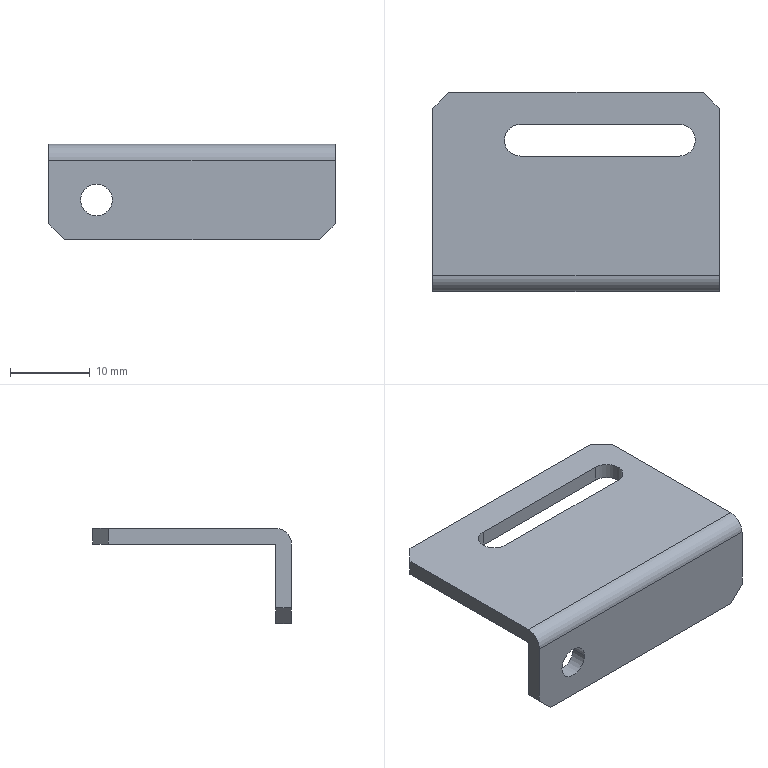Component | SolidWorks | WirePressingUnitFiberOpticBracket-1 | 1 solid | 20 faces | box 36 x 25 x 12 mm | volume 2263 mm3 | plane 14 | cylinder 6 | commonest cylinder face diameters 4 x6
build123d program:
from build123d import *

# Parameters (mm, degrees)
BOSS_EXTRUDE1_DEPTH = 18
M4_TAPPED_HOLE1_D   = 4
CHAMFER1_SIZE       = 2
CUT_EXTRUDE1_DEPTH  = 10


with BuildPart() as part:
    # Sketch1 → Boss-Extrude1 (new, symmetric)
    with BuildSketch(Plane.XY):
        with BuildLine():
            Line((0, 0), (10, 0))
            ThreePointArc((10, 0), (11.414, 0.5858), (12, 2))
            Line((12, 2), (12, 25))
            Line((12, 25), (10, 25))
            Line((10, 25), (10, 2))
            Line((10, 2), (0, 2))
            Line((0, 2), (0, 0))
        make_face()
    extrude(amount=BOSS_EXTRUDE1_DEPTH, both=True)

    # M4 Tapped Hole1 (through all)
    with Locations(Plane(origin=(0, 0, 0), x_dir=(-1, 0, 0), z_dir=(0, -1, 0))):
        with Locations((-5, -12)):
            Hole(M4_TAPPED_HOLE1_D / 2)

    # Chamfer1
    chamfer1_edges = [part.edges().sort_by_distance(p)[0] for p in [
        (11, 25, 18),
        (0, 1, 18),
        (11, 25, -18),
        (0, 1, -18),
    ]]
    chamfer(chamfer1_edges, length=CHAMFER1_SIZE)

    # Sketch4 → Cut-Extrude1 (cut)
    with BuildSketch(Plane.ZY.offset(-10)):
        with BuildLine():
            Line((-13, 21), (7, 21))
            ThreePointArc((7, 21), (9, 19), (7, 17))
            Line((7, 17), (-13, 17))
            ThreePointArc((-13, 17), (-15, 19), (-13, 21))
        make_face()
    extrude(amount=-CUT_EXTRUDE1_DEPTH, mode=Mode.SUBTRACT)


solid = part.part

# Placed as in the assembly
solid = solid.moved(Location((32.665, -6.632, -220.315), (0, -90, 0)))
STEP:
#1=COLOUR_RGB('',0.7922,0.8196,0.9333);
#2=FILL_AREA_STYLE_COLOUR('',#1);
#3=FILL_AREA_STYLE('',(#2));
#4=SURFACE_STYLE_FILL_AREA(#3);
#5=SURFACE_SIDE_STYLE('',(#4));
#6=SURFACE_STYLE_USAGE(.BOTH.,#5);
#7=PRESENTATION_STYLE_ASSIGNMENT((#6));
#8=CARTESIAN_POINT('',(0.9317,0.4869,-8.201));
#9=VERTEX_POINT('',#8);
#10=CARTESIAN_POINT('',(1.01,0.5657,-8.201));
#11=VERTEX_POINT('',#10);
#12=CARTESIAN_POINT('',(1.01,0.4869,-8.201));
#13=DIRECTION('',(-0.,0.,-1.));
#14=DIRECTION('',(0.,-1.,0.));
#15=AXIS2_PLACEMENT_3D('',#12,#13,#14);
#16=CIRCLE('',#15,0.07874);
#17=EDGE_CURVE('',#9,#11,#16,.T.);
#18=ORIENTED_EDGE('',*,*,#17,.F.);
#19=CARTESIAN_POINT('',(0.9317,0.4869,-8.28));
#20=VERTEX_POINT('',#19);
#21=CARTESIAN_POINT('',(0.9317,0.4869,-7.886));
#22=DIRECTION('',(-0.,-0.,-1.));
#23=VECTOR('',#22,39.37);
#24=LINE('',#21,#23);
#25=EDGE_CURVE('',#9,#20,#24,.T.);
#26=ORIENTED_EDGE('',*,*,#25,.T.);
#27=CARTESIAN_POINT('',(1.01,0.5657,-8.28));
#28=VERTEX_POINT('',#27);
#29=CARTESIAN_POINT('',(1.01,0.4869,-8.28));
#30=DIRECTION('',(-0.,-0.,-1.));
#31=DIRECTION('',(-1.,0.,0.));
#32=AXIS2_PLACEMENT_3D('',#29,#30,#31);
#33=CIRCLE('',#32,0.07874);
#34=EDGE_CURVE('',#20,#28,#33,.T.);
#35=ORIENTED_EDGE('',*,*,#34,.T.);
#36=CARTESIAN_POINT('',(1.01,0.5657,-7.886));
#37=DIRECTION('',(-0.,-0.,-1.));
#38=VECTOR('',#37,39.37);
#39=LINE('',#36,#38);
#40=EDGE_CURVE('',#11,#28,#39,.T.);
#41=ORIENTED_EDGE('',*,*,#40,.F.);
#42=EDGE_LOOP('',(#18,#26,#35,#41));
#43=FACE_OUTER_BOUND('',#42,.T.);
#44=CARTESIAN_POINT('',(1.01,0.4869,-7.886));
#45=DIRECTION('',(-0.,-0.,-1.));
#46=DIRECTION('',(-1.,0.,0.));
#47=AXIS2_PLACEMENT_3D('',#44,#45,#46);
#48=CYLINDRICAL_SURFACE('',#47,0.07874);
#49=ADVANCED_FACE('',(#43),#48,.F.);
#50=CARTESIAN_POINT('',(0.7348,-0.1824,-8.477));
#51=VERTEX_POINT('',#50);
#52=CARTESIAN_POINT('',(0.8923,-0.1824,-8.477));
#53=VERTEX_POINT('',#52);
#54=CARTESIAN_POINT('',(0.8136,-0.1824,-8.477));
#55=DIRECTION('',(-0.,-1.,-0.));
#56=DIRECTION('',(1.,0.,0.));
#57=AXIS2_PLACEMENT_3D('',#54,#55,#56);
#58=CIRCLE('',#57,0.07874);
#59=EDGE_CURVE('',#51,#53,#58,.T.);
#60=ORIENTED_EDGE('',*,*,#59,.F.);
#61=CARTESIAN_POINT('',(0.7348,-0.2611,-8.477));
#62=VERTEX_POINT('',#61);
#63=CARTESIAN_POINT('',(0.7348,-0.2611,-8.477));
#64=DIRECTION('',(-0.,-1.,-0.));
#65=VECTOR('',#64,39.37);
#66=LINE('',#63,#65);
#67=EDGE_CURVE('',#51,#62,#66,.T.);
#68=ORIENTED_EDGE('',*,*,#67,.T.);
#69=CARTESIAN_POINT('',(0.8923,-0.2611,-8.477));
#70=VERTEX_POINT('',#69);
#71=CARTESIAN_POINT('',(0.8136,-0.2611,-8.477));
#72=DIRECTION('',(-0.,-1.,-0.));
#73=DIRECTION('',(1.,0.,0.));
#74=AXIS2_PLACEMENT_3D('',#71,#72,#73);
#75=CIRCLE('',#74,0.07874);
#76=EDGE_CURVE('',#62,#70,#75,.T.);
#77=ORIENTED_EDGE('',*,*,#76,.T.);
#78=CARTESIAN_POINT('',(0.8923,-0.2611,-8.477));
#79=DIRECTION('',(-0.,-1.,-0.));
#80=VECTOR('',#79,39.37);
#81=LINE('',#78,#80);
#82=EDGE_CURVE('',#53,#70,#81,.T.);
#83=ORIENTED_EDGE('',*,*,#82,.F.);
#84=EDGE_LOOP('',(#60,#68,#77,#83));
#85=FACE_OUTER_BOUND('',#84,.T.);
#86=CARTESIAN_POINT('',(0.8136,-0.2611,-8.477));
#87=DIRECTION('',(-0.,-1.,-0.));
#88=DIRECTION('',(1.,0.,0.));
#89=AXIS2_PLACEMENT_3D('',#86,#87,#88);
#90=CYLINDRICAL_SURFACE('',#89,0.07874);
#91=ADVANCED_FACE('',(#85),#90,.F.);
#92=CARTESIAN_POINT('',(0.6561,-0.1824,-8.674));
#93=VERTEX_POINT('',#92);
#94=CARTESIAN_POINT('',(1.916,-0.1824,-8.674));
#95=VERTEX_POINT('',#94);
#96=CARTESIAN_POINT('',(0.5774,-0.1824,-8.674));
#97=DIRECTION('',(1.,0.,-0.));
#98=VECTOR('',#97,39.37);
#99=LINE('',#96,#98);
#100=EDGE_CURVE('',#93,#95,#99,.T.);
#101=ORIENTED_EDGE('',*,*,#100,.T.);
#102=CARTESIAN_POINT('',(1.916,-0.2611,-8.674));
#103=VERTEX_POINT('',#102);
#104=CARTESIAN_POINT('',(1.916,-0.1824,-8.674));
#105=DIRECTION('',(-0.,-1.,-0.));
#106=VECTOR('',#105,39.37);
#107=LINE('',#104,#106);
#108=EDGE_CURVE('',#95,#103,#107,.T.);
#109=ORIENTED_EDGE('',*,*,#108,.T.);
#110=CARTESIAN_POINT('',(0.6561,-0.2611,-8.674));
#111=VERTEX_POINT('',#110);
#112=CARTESIAN_POINT('',(0.5774,-0.2611,-8.674));
#113=DIRECTION('',(1.,0.,-0.));
#114=VECTOR('',#113,39.37);
#115=LINE('',#112,#114);
#116=EDGE_CURVE('',#111,#103,#115,.T.);
#117=ORIENTED_EDGE('',*,*,#116,.F.);
#118=CARTESIAN_POINT('',(0.6561,-0.1824,-8.674));
#119=DIRECTION('',(0.,1.,0.));
#120=VECTOR('',#119,39.37);
#121=LINE('',#118,#120);
#122=EDGE_CURVE('',#111,#93,#121,.T.);
#123=ORIENTED_EDGE('',*,*,#122,.T.);
#124=EDGE_LOOP('',(#101,#109,#117,#123));
#125=FACE_OUTER_BOUND('',#124,.T.);
#126=CARTESIAN_POINT('',(0.5774,-0.1824,-8.674));
#127=DIRECTION('',(0.,0.,1.));
#128=DIRECTION('',(1.,0.,-0.));
#129=AXIS2_PLACEMENT_3D('',#126,#127,#128);
#130=PLANE('',#129);
#131=ADVANCED_FACE('',(#125),#130,.F.);
#132=CARTESIAN_POINT('',(0.8136,-0.2611,-8.477));
#133=DIRECTION('',(-0.,-1.,-0.));
#134=DIRECTION('',(1.,0.,0.));
#135=AXIS2_PLACEMENT_3D('',#132,#133,#134);
#136=CIRCLE('',#135,0.07874);
#137=EDGE_CURVE('',#70,#62,#136,.T.);
#138=ORIENTED_EDGE('',*,*,#137,.F.);
#139=ORIENTED_EDGE('',*,*,#76,.F.);
#140=EDGE_LOOP('',(#138,#139));
#141=FACE_BOUND('',#140,.T.);
#142=ORIENTED_EDGE('',*,*,#116,.T.);
#143=CARTESIAN_POINT('',(1.995,-0.2611,-8.595));
#144=VERTEX_POINT('',#143);
#145=CARTESIAN_POINT('',(1.916,-0.2611,-8.674));
#146=DIRECTION('',(0.7071,0.,0.7071));
#147=VECTOR('',#146,39.37);
#148=LINE('',#145,#147);
#149=EDGE_CURVE('',#103,#144,#148,.T.);
#150=ORIENTED_EDGE('',*,*,#149,.T.);
#151=CARTESIAN_POINT('',(1.995,-0.2611,-8.28));
#152=VERTEX_POINT('',#151);
#153=CARTESIAN_POINT('',(1.995,-0.2611,-8.674));
#154=DIRECTION('',(0.,0.,1.));
#155=VECTOR('',#154,39.37);
#156=LINE('',#153,#155);
#157=EDGE_CURVE('',#144,#152,#156,.T.);
#158=ORIENTED_EDGE('',*,*,#157,.T.);
#159=CARTESIAN_POINT('',(0.5774,-0.2611,-8.28));
#160=VERTEX_POINT('',#159);
#161=CARTESIAN_POINT('',(0.5774,-0.2611,-8.28));
#162=DIRECTION('',(1.,0.,-0.));
#163=VECTOR('',#162,39.37);
#164=LINE('',#161,#163);
#165=EDGE_CURVE('',#160,#152,#164,.T.);
#166=ORIENTED_EDGE('',*,*,#165,.F.);
#167=CARTESIAN_POINT('',(0.5774,-0.2611,-8.595));
#168=VERTEX_POINT('',#167);
#169=CARTESIAN_POINT('',(0.5774,-0.2611,-8.674));
#170=DIRECTION('',(0.,0.,1.));
#171=VECTOR('',#170,39.37);
#172=LINE('',#169,#171);
#173=EDGE_CURVE('',#168,#160,#172,.T.);
#174=ORIENTED_EDGE('',*,*,#173,.F.);
#175=CARTESIAN_POINT('',(0.5774,-0.2611,-8.595));
#176=DIRECTION('',(0.7071,-0.,-0.7071));
#177=VECTOR('',#176,39.37);
#178=LINE('',#175,#177);
#179=EDGE_CURVE('',#168,#111,#178,.T.);
#180=ORIENTED_EDGE('',*,*,#179,.T.);
#181=EDGE_LOOP('',(#142,#150,#158,#166,#174,#180));
#182=FACE_OUTER_BOUND('',#181,.T.);
#183=CARTESIAN_POINT('',(0.5774,-0.2611,-8.674));
#184=DIRECTION('',(-0.,1.,0.));
#185=DIRECTION('',(-1.,-0.,0.));
#186=AXIS2_PLACEMENT_3D('',#183,#184,#185);
#187=PLANE('',#186);
#188=ADVANCED_FACE('',(#141,#182),#187,.F.);
#189=CARTESIAN_POINT('',(1.995,-0.1824,-8.201));
#190=VERTEX_POINT('',#189);
#191=CARTESIAN_POINT('',(1.995,-0.1824,-8.28));
#192=DIRECTION('',(-1.,-0.,0.));
#193=DIRECTION('',(0.,0.,1.));
#194=AXIS2_PLACEMENT_3D('',#191,#192,#193);
#195=CIRCLE('',#194,0.07874);
#196=EDGE_CURVE('',#152,#190,#195,.T.);
#197=ORIENTED_EDGE('',*,*,#196,.T.);
#198=CARTESIAN_POINT('',(0.5774,-0.1824,-8.201));
#199=VERTEX_POINT('',#198);
#200=CARTESIAN_POINT('',(0.5774,-0.1824,-8.201));
#201=DIRECTION('',(1.,0.,-0.));
#202=VECTOR('',#201,39.37);
#203=LINE('',#200,#202);
#204=EDGE_CURVE('',#199,#190,#203,.T.);
#205=ORIENTED_EDGE('',*,*,#204,.F.);
#206=CARTESIAN_POINT('',(0.5774,-0.1824,-8.28));
#207=DIRECTION('',(-1.,-0.,0.));
#208=DIRECTION('',(0.,0.,1.));
#209=AXIS2_PLACEMENT_3D('',#206,#207,#208);
#210=CIRCLE('',#209,0.07874);
#211=EDGE_CURVE('',#160,#199,#210,.T.);
#212=ORIENTED_EDGE('',*,*,#211,.F.);
#213=ORIENTED_EDGE('',*,*,#165,.T.);
#214=EDGE_LOOP('',(#197,#205,#212,#213));
#215=FACE_OUTER_BOUND('',#214,.T.);
#216=CARTESIAN_POINT('',(0.5774,-0.1824,-8.28));
#217=DIRECTION('',(1.,0.,-0.));
#218=DIRECTION('',(0.,0.,-1.));
#219=AXIS2_PLACEMENT_3D('',#216,#217,#218);
#220=CYLINDRICAL_SURFACE('',#219,0.07874);
#221=ADVANCED_FACE('',(#215),#220,.T.);
#222=CARTESIAN_POINT('',(1.798,0.5657,-8.201));
#223=VERTEX_POINT('',#222);
#224=CARTESIAN_POINT('',(0.5774,0.5657,-8.201));
#225=DIRECTION('',(1.,0.,-0.));
#226=VECTOR('',#225,39.37);
#227=LINE('',#224,#226);
#228=EDGE_CURVE('',#11,#223,#227,.T.);
#229=ORIENTED_EDGE('',*,*,#228,.T.);
#230=CARTESIAN_POINT('',(1.798,0.4082,-8.201));
#231=VERTEX_POINT('',#230);
#232=CARTESIAN_POINT('',(1.798,0.4869,-8.201));
#233=DIRECTION('',(-0.,0.,-1.));
#234=DIRECTION('',(0.,-1.,0.));
#235=AXIS2_PLACEMENT_3D('',#232,#233,#234);
#236=CIRCLE('',#235,0.07874);
#237=EDGE_CURVE('',#223,#231,#236,.T.);
#238=ORIENTED_EDGE('',*,*,#237,.T.);
#239=CARTESIAN_POINT('',(1.01,0.4082,-8.201));
#240=VERTEX_POINT('',#239);
#241=CARTESIAN_POINT('',(0.5774,0.4082,-8.201));
#242=DIRECTION('',(-1.,-0.,0.));
#243=VECTOR('',#242,39.37);
#244=LINE('',#241,#243);
#245=EDGE_CURVE('',#231,#240,#244,.T.);
#246=ORIENTED_EDGE('',*,*,#245,.T.);
#247=CARTESIAN_POINT('',(1.01,0.4869,-8.201));
#248=DIRECTION('',(-0.,0.,-1.));
#249=DIRECTION('',(0.,-1.,0.));
#250=AXIS2_PLACEMENT_3D('',#247,#248,#249);
#251=CIRCLE('',#250,0.07874);
#252=EDGE_CURVE('',#240,#9,#251,.T.);
#253=ORIENTED_EDGE('',*,*,#252,.T.);
#254=ORIENTED_EDGE('',*,*,#17,.T.);
#255=EDGE_LOOP('',(#229,#238,#246,#253,#254));
#256=FACE_BOUND('',#255,.T.);
#257=CARTESIAN_POINT('',(0.6561,0.7232,-8.201));
#258=VERTEX_POINT('',#257);
#259=CARTESIAN_POINT('',(1.916,0.7232,-8.201));
#260=VERTEX_POINT('',#259);
#261=CARTESIAN_POINT('',(0.5774,0.7232,-8.201));
#262=DIRECTION('',(1.,0.,-0.));
#263=VECTOR('',#262,39.37);
#264=LINE('',#261,#263);
#265=EDGE_CURVE('',#258,#260,#264,.T.);
#266=ORIENTED_EDGE('',*,*,#265,.F.);
#267=CARTESIAN_POINT('',(0.5774,0.6444,-8.201));
#268=VERTEX_POINT('',#267);
#269=CARTESIAN_POINT('',(0.5774,0.6444,-8.201));
#270=DIRECTION('',(-0.7071,-0.7071,0.));
#271=VECTOR('',#270,39.37);
#272=LINE('',#269,#271);
#273=EDGE_CURVE('',#258,#268,#272,.T.);
#274=ORIENTED_EDGE('',*,*,#273,.T.);
#275=CARTESIAN_POINT('',(0.5774,-0.1824,-8.201));
#276=DIRECTION('',(0.,1.,0.));
#277=VECTOR('',#276,39.37);
#278=LINE('',#275,#277);
#279=EDGE_CURVE('',#199,#268,#278,.T.);
#280=ORIENTED_EDGE('',*,*,#279,.F.);
#281=ORIENTED_EDGE('',*,*,#204,.T.);
#282=CARTESIAN_POINT('',(1.995,0.6444,-8.201));
#283=VERTEX_POINT('',#282);
#284=CARTESIAN_POINT('',(1.995,-0.1824,-8.201));
#285=DIRECTION('',(0.,1.,0.));
#286=VECTOR('',#285,39.37);
#287=LINE('',#284,#286);
#288=EDGE_CURVE('',#190,#283,#287,.T.);
#289=ORIENTED_EDGE('',*,*,#288,.T.);
#290=CARTESIAN_POINT('',(1.916,0.7232,-8.201));
#291=DIRECTION('',(-0.7071,0.7071,0.));
#292=VECTOR('',#291,39.37);
#293=LINE('',#290,#292);
#294=EDGE_CURVE('',#283,#260,#293,.T.);
#295=ORIENTED_EDGE('',*,*,#294,.T.);
#296=EDGE_LOOP('',(#266,#274,#280,#281,#289,#295));
#297=FACE_OUTER_BOUND('',#296,.T.);
#298=CARTESIAN_POINT('',(0.5774,-0.1824,-8.201));
#299=DIRECTION('',(-0.,0.,-1.));
#300=DIRECTION('',(-0.,-1.,-0.));
#301=AXIS2_PLACEMENT_3D('',#298,#299,#300);
#302=PLANE('',#301);
#303=ADVANCED_FACE('',(#256,#297),#302,.F.);
#304=CARTESIAN_POINT('',(0.6561,0.7232,-8.28));
#305=VERTEX_POINT('',#304);
#306=CARTESIAN_POINT('',(1.916,0.7232,-8.28));
#307=VERTEX_POINT('',#306);
#308=CARTESIAN_POINT('',(0.5774,0.7232,-8.28));
#309=DIRECTION('',(1.,0.,-0.));
#310=VECTOR('',#309,39.37);
#311=LINE('',#308,#310);
#312=EDGE_CURVE('',#305,#307,#311,.T.);
#313=ORIENTED_EDGE('',*,*,#312,.F.);
#314=CARTESIAN_POINT('',(0.6561,0.7232,-8.201));
#315=DIRECTION('',(0.,0.,1.));
#316=VECTOR('',#315,39.37);
#317=LINE('',#314,#316);
#318=EDGE_CURVE('',#305,#258,#317,.T.);
#319=ORIENTED_EDGE('',*,*,#318,.T.);
#320=ORIENTED_EDGE('',*,*,#265,.T.);
#321=CARTESIAN_POINT('',(1.916,0.7232,-8.28));
#322=DIRECTION('',(-0.,-0.,-1.));
#323=VECTOR('',#322,39.37);
#324=LINE('',#321,#323);
#325=EDGE_CURVE('',#260,#307,#324,.T.);
#326=ORIENTED_EDGE('',*,*,#325,.T.);
#327=EDGE_LOOP('',(#313,#319,#320,#326));
#328=FACE_OUTER_BOUND('',#327,.T.);
#329=CARTESIAN_POINT('',(0.5774,0.7232,-8.28));
#330=DIRECTION('',(0.,-1.,-0.));
#331=DIRECTION('',(1.,0.,-0.));
#332=AXIS2_PLACEMENT_3D('',#329,#330,#331);
#333=PLANE('',#332);
#334=ADVANCED_FACE('',(#328),#333,.F.);
#335=CARTESIAN_POINT('',(1.798,0.4082,-8.28));
#336=VERTEX_POINT('',#335);
#337=CARTESIAN_POINT('',(1.01,0.4082,-8.28));
#338=VERTEX_POINT('',#337);
#339=CARTESIAN_POINT('',(1.798,0.4082,-8.28));
#340=DIRECTION('',(-1.,-0.,0.));
#341=VECTOR('',#340,39.37);
#342=LINE('',#339,#341);
#343=EDGE_CURVE('',#336,#338,#342,.T.);
#344=ORIENTED_EDGE('',*,*,#343,.F.);
#345=CARTESIAN_POINT('',(1.798,0.5657,-8.28));
#346=VERTEX_POINT('',#345);
#347=CARTESIAN_POINT('',(1.798,0.4869,-8.28));
#348=DIRECTION('',(-0.,-0.,-1.));
#349=DIRECTION('',(-1.,0.,0.));
#350=AXIS2_PLACEMENT_3D('',#347,#348,#349);
#351=CIRCLE('',#350,0.07874);
#352=EDGE_CURVE('',#346,#336,#351,.T.);
#353=ORIENTED_EDGE('',*,*,#352,.F.);
#354=CARTESIAN_POINT('',(1.798,0.5657,-8.28));
#355=DIRECTION('',(1.,0.,-0.));
#356=VECTOR('',#355,39.37);
#357=LINE('',#354,#356);
#358=EDGE_CURVE('',#28,#346,#357,.T.);
#359=ORIENTED_EDGE('',*,*,#358,.F.);
#360=ORIENTED_EDGE('',*,*,#34,.F.);
#361=CARTESIAN_POINT('',(1.01,0.4869,-8.28));
#362=DIRECTION('',(-0.,-0.,-1.));
#363=DIRECTION('',(-1.,0.,0.));
#364=AXIS2_PLACEMENT_3D('',#361,#362,#363);
#365=CIRCLE('',#364,0.07874);
#366=EDGE_CURVE('',#338,#20,#365,.T.);
#367=ORIENTED_EDGE('',*,*,#366,.F.);
#368=EDGE_LOOP('',(#344,#353,#359,#360,#367));
#369=FACE_BOUND('',#368,.T.);
#370=CARTESIAN_POINT('',(0.5774,0.6444,-8.28));
#371=VERTEX_POINT('',#370);
#372=CARTESIAN_POINT('',(0.5774,-0.1824,-8.28));
#373=VERTEX_POINT('',#372);
#374=CARTESIAN_POINT('',(0.5774,-0.1824,-8.28));
#375=DIRECTION('',(-0.,-1.,-0.));
#376=VECTOR('',#375,39.37);
#377=LINE('',#374,#376);
#378=EDGE_CURVE('',#371,#373,#377,.T.);
#379=ORIENTED_EDGE('',*,*,#378,.F.);
#380=CARTESIAN_POINT('',(0.5774,0.6444,-8.28));
#381=DIRECTION('',(0.7071,0.7071,-0.));
#382=VECTOR('',#381,39.37);
#383=LINE('',#380,#382);
#384=EDGE_CURVE('',#371,#305,#383,.T.);
#385=ORIENTED_EDGE('',*,*,#384,.T.);
#386=ORIENTED_EDGE('',*,*,#312,.T.);
#387=CARTESIAN_POINT('',(1.995,0.6444,-8.28));
#388=VERTEX_POINT('',#387);
#389=CARTESIAN_POINT('',(1.916,0.7232,-8.28));
#390=DIRECTION('',(0.7071,-0.7071,-0.));
#391=VECTOR('',#390,39.37);
#392=LINE('',#389,#391);
#393=EDGE_CURVE('',#307,#388,#392,.T.);
#394=ORIENTED_EDGE('',*,*,#393,.T.);
#395=CARTESIAN_POINT('',(1.995,-0.1824,-8.28));
#396=VERTEX_POINT('',#395);
#397=CARTESIAN_POINT('',(1.995,-0.1824,-8.28));
#398=DIRECTION('',(-0.,-1.,-0.));
#399=VECTOR('',#398,39.37);
#400=LINE('',#397,#399);
#401=EDGE_CURVE('',#388,#396,#400,.T.);
#402=ORIENTED_EDGE('',*,*,#401,.T.);
#403=CARTESIAN_POINT('',(0.5774,-0.1824,-8.28));
#404=DIRECTION('',(1.,0.,-0.));
#405=VECTOR('',#404,39.37);
#406=LINE('',#403,#405);
#407=EDGE_CURVE('',#373,#396,#406,.T.);
#408=ORIENTED_EDGE('',*,*,#407,.F.);
#409=EDGE_LOOP('',(#379,#385,#386,#394,#402,#408));
#410=FACE_OUTER_BOUND('',#409,.T.);
#411=CARTESIAN_POINT('',(0.5774,-0.1824,-8.28));
#412=DIRECTION('',(0.,0.,1.));
#413=DIRECTION('',(1.,0.,-0.));
#414=AXIS2_PLACEMENT_3D('',#411,#412,#413);
#415=PLANE('',#414);
#416=ADVANCED_FACE('',(#369,#410),#415,.F.);
#417=CARTESIAN_POINT('',(0.8136,-0.1824,-8.477));
#418=DIRECTION('',(-0.,-1.,-0.));
#419=DIRECTION('',(1.,0.,0.));
#420=AXIS2_PLACEMENT_3D('',#417,#418,#419);
#421=CIRCLE('',#420,0.07874);
#422=EDGE_CURVE('',#53,#51,#421,.T.);
#423=ORIENTED_EDGE('',*,*,#422,.T.);
#424=ORIENTED_EDGE('',*,*,#59,.T.);
#425=EDGE_LOOP('',(#423,#424));
#426=FACE_BOUND('',#425,.T.);
#427=CARTESIAN_POINT('',(1.995,-0.1824,-8.595));
#428=VERTEX_POINT('',#427);
#429=CARTESIAN_POINT('',(1.995,-0.1824,-8.674));
#430=DIRECTION('',(-0.,-0.,-1.));
#431=VECTOR('',#430,39.37);
#432=LINE('',#429,#431);
#433=EDGE_CURVE('',#396,#428,#432,.T.);
#434=ORIENTED_EDGE('',*,*,#433,.T.);
#435=CARTESIAN_POINT('',(1.916,-0.1824,-8.674));
#436=DIRECTION('',(-0.7071,-0.,-0.7071));
#437=VECTOR('',#436,39.37);
#438=LINE('',#435,#437);
#439=EDGE_CURVE('',#428,#95,#438,.T.);
#440=ORIENTED_EDGE('',*,*,#439,.T.);
#441=ORIENTED_EDGE('',*,*,#100,.F.);
#442=CARTESIAN_POINT('',(0.5774,-0.1824,-8.595));
#443=VERTEX_POINT('',#442);
#444=CARTESIAN_POINT('',(0.5774,-0.1824,-8.595));
#445=DIRECTION('',(-0.7071,0.,0.7071));
#446=VECTOR('',#445,39.37);
#447=LINE('',#444,#446);
#448=EDGE_CURVE('',#93,#443,#447,.T.);
#449=ORIENTED_EDGE('',*,*,#448,.T.);
#450=CARTESIAN_POINT('',(0.5774,-0.1824,-8.674));
#451=DIRECTION('',(-0.,-0.,-1.));
#452=VECTOR('',#451,39.37);
#453=LINE('',#450,#452);
#454=EDGE_CURVE('',#373,#443,#453,.T.);
#455=ORIENTED_EDGE('',*,*,#454,.F.);
#456=ORIENTED_EDGE('',*,*,#407,.T.);
#457=EDGE_LOOP('',(#434,#440,#441,#449,#455,#456));
#458=FACE_OUTER_BOUND('',#457,.T.);
#459=CARTESIAN_POINT('',(0.5774,-0.1824,-8.674));
#460=DIRECTION('',(0.,-1.,-0.));
#461=DIRECTION('',(1.,0.,-0.));
#462=AXIS2_PLACEMENT_3D('',#459,#460,#461);
#463=PLANE('',#462);
#464=ADVANCED_FACE('',(#426,#458),#463,.F.);
#465=ORIENTED_EDGE('',*,*,#279,.T.);
#466=CARTESIAN_POINT('',(0.5774,0.6444,-8.28));
#467=DIRECTION('',(-0.,-0.,-1.));
#468=VECTOR('',#467,39.37);
#469=LINE('',#466,#468);
#470=EDGE_CURVE('',#268,#371,#469,.T.);
#471=ORIENTED_EDGE('',*,*,#470,.T.);
#472=ORIENTED_EDGE('',*,*,#378,.T.);
#473=ORIENTED_EDGE('',*,*,#454,.T.);
#474=CARTESIAN_POINT('',(0.5774,-0.2611,-8.595));
#475=DIRECTION('',(-0.,-1.,-0.));
#476=VECTOR('',#475,39.37);
#477=LINE('',#474,#476);
#478=EDGE_CURVE('',#443,#168,#477,.T.);
#479=ORIENTED_EDGE('',*,*,#478,.T.);
#480=ORIENTED_EDGE('',*,*,#173,.T.);
#481=ORIENTED_EDGE('',*,*,#211,.T.);
#482=EDGE_LOOP('',(#465,#471,#472,#473,#479,#480,#481));
#483=FACE_OUTER_BOUND('',#482,.T.);
#484=CARTESIAN_POINT('',(0.5774,-0.1824,-8.28));
#485=DIRECTION('',(-1.,-0.,0.));
#486=DIRECTION('',(0.,0.,1.));
#487=AXIS2_PLACEMENT_3D('',#484,#485,#486);
#488=PLANE('',#487);
#489=ADVANCED_FACE('',(#483),#488,.T.);
#490=ORIENTED_EDGE('',*,*,#401,.F.);
#491=CARTESIAN_POINT('',(1.995,0.6444,-8.28));
#492=DIRECTION('',(0.,0.,1.));
#493=VECTOR('',#492,39.37);
#494=LINE('',#491,#493);
#495=EDGE_CURVE('',#388,#283,#494,.T.);
#496=ORIENTED_EDGE('',*,*,#495,.T.);
#497=ORIENTED_EDGE('',*,*,#288,.F.);
#498=ORIENTED_EDGE('',*,*,#196,.F.);
#499=ORIENTED_EDGE('',*,*,#157,.F.);
#500=CARTESIAN_POINT('',(1.995,-0.1824,-8.595));
#501=DIRECTION('',(0.,1.,0.));
#502=VECTOR('',#501,39.37);
#503=LINE('',#500,#502);
#504=EDGE_CURVE('',#144,#428,#503,.T.);
#505=ORIENTED_EDGE('',*,*,#504,.T.);
#506=ORIENTED_EDGE('',*,*,#433,.F.);
#507=EDGE_LOOP('',(#490,#496,#497,#498,#499,#505,#506));
#508=FACE_OUTER_BOUND('',#507,.T.);
#509=CARTESIAN_POINT('',(1.995,-0.1824,-8.28));
#510=DIRECTION('',(-1.,-0.,0.));
#511=DIRECTION('',(0.,0.,1.));
#512=AXIS2_PLACEMENT_3D('',#509,#510,#511);
#513=PLANE('',#512);
#514=ADVANCED_FACE('',(#508),#513,.F.);
#515=ORIENTED_EDGE('',*,*,#67,.F.);
#516=ORIENTED_EDGE('',*,*,#422,.F.);
#517=ORIENTED_EDGE('',*,*,#82,.T.);
#518=ORIENTED_EDGE('',*,*,#137,.T.);
#519=EDGE_LOOP('',(#515,#516,#517,#518));
#520=FACE_OUTER_BOUND('',#519,.T.);
#521=CARTESIAN_POINT('',(0.8136,-0.2611,-8.477));
#522=DIRECTION('',(-0.,-1.,-0.));
#523=DIRECTION('',(1.,0.,0.));
#524=AXIS2_PLACEMENT_3D('',#521,#522,#523);
#525=CYLINDRICAL_SURFACE('',#524,0.07874);
#526=ADVANCED_FACE('',(#520),#525,.F.);
#527=ORIENTED_EDGE('',*,*,#273,.F.);
#528=ORIENTED_EDGE('',*,*,#318,.F.);
#529=ORIENTED_EDGE('',*,*,#384,.F.);
#530=ORIENTED_EDGE('',*,*,#470,.F.);
#531=EDGE_LOOP('',(#527,#528,#529,#530));
#532=FACE_OUTER_BOUND('',#531,.T.);
#533=CARTESIAN_POINT('',(0.5774,0.6444,-8.28));
#534=DIRECTION('',(-0.7071,0.7071,0.));
#535=DIRECTION('',(0.,0.,1.));
#536=AXIS2_PLACEMENT_3D('',#533,#534,#535);
#537=PLANE('',#536);
#538=ADVANCED_FACE('',(#532),#537,.T.);
#539=ORIENTED_EDGE('',*,*,#294,.F.);
#540=ORIENTED_EDGE('',*,*,#495,.F.);
#541=ORIENTED_EDGE('',*,*,#393,.F.);
#542=ORIENTED_EDGE('',*,*,#325,.F.);
#543=EDGE_LOOP('',(#539,#540,#541,#542));
#544=FACE_OUTER_BOUND('',#543,.T.);
#545=CARTESIAN_POINT('',(1.916,0.7232,-8.28));
#546=DIRECTION('',(-0.7071,-0.7071,0.));
#547=DIRECTION('',(-0.,-0.,-1.));
#548=AXIS2_PLACEMENT_3D('',#545,#546,#547);
#549=PLANE('',#548);
#550=ADVANCED_FACE('',(#544),#549,.F.);
#551=ORIENTED_EDGE('',*,*,#439,.F.);
#552=ORIENTED_EDGE('',*,*,#504,.F.);
#553=ORIENTED_EDGE('',*,*,#149,.F.);
#554=ORIENTED_EDGE('',*,*,#108,.F.);
#555=EDGE_LOOP('',(#551,#552,#553,#554));
#556=FACE_OUTER_BOUND('',#555,.T.);
#557=CARTESIAN_POINT('',(1.916,-0.1824,-8.674));
#558=DIRECTION('',(-0.7071,-0.,0.7071));
#559=DIRECTION('',(-0.,-1.,-0.));
#560=AXIS2_PLACEMENT_3D('',#557,#558,#559);
#561=PLANE('',#560);
#562=ADVANCED_FACE('',(#556),#561,.F.);
#563=ORIENTED_EDGE('',*,*,#448,.F.);
#564=ORIENTED_EDGE('',*,*,#122,.F.);
#565=ORIENTED_EDGE('',*,*,#179,.F.);
#566=ORIENTED_EDGE('',*,*,#478,.F.);
#567=EDGE_LOOP('',(#563,#564,#565,#566));
#568=FACE_OUTER_BOUND('',#567,.T.);
#569=CARTESIAN_POINT('',(0.5774,-0.1824,-8.595));
#570=DIRECTION('',(-0.7071,0.,-0.7071));
#571=DIRECTION('',(0.,1.,0.));
#572=AXIS2_PLACEMENT_3D('',#569,#570,#571);
#573=PLANE('',#572);
#574=ADVANCED_FACE('',(#568),#573,.T.);
#575=CARTESIAN_POINT('',(1.798,0.5657,-7.886));
#576=DIRECTION('',(-0.,-0.,-1.));
#577=VECTOR('',#576,39.37);
#578=LINE('',#575,#577);
#579=EDGE_CURVE('',#223,#346,#578,.T.);
#580=ORIENTED_EDGE('',*,*,#579,.T.);
#581=ORIENTED_EDGE('',*,*,#352,.T.);
#582=CARTESIAN_POINT('',(1.798,0.4082,-7.886));
#583=DIRECTION('',(-0.,-0.,-1.));
#584=VECTOR('',#583,39.37);
#585=LINE('',#582,#584);
#586=EDGE_CURVE('',#231,#336,#585,.T.);
#587=ORIENTED_EDGE('',*,*,#586,.F.);
#588=ORIENTED_EDGE('',*,*,#237,.F.);
#589=EDGE_LOOP('',(#580,#581,#587,#588));
#590=FACE_OUTER_BOUND('',#589,.T.);
#591=CARTESIAN_POINT('',(1.798,0.4869,-7.886));
#592=DIRECTION('',(-0.,-0.,-1.));
#593=DIRECTION('',(-1.,0.,0.));
#594=AXIS2_PLACEMENT_3D('',#591,#592,#593);
#595=CYLINDRICAL_SURFACE('',#594,0.07874);
#596=ADVANCED_FACE('',(#590),#595,.F.);
#597=ORIENTED_EDGE('',*,*,#40,.T.);
#598=ORIENTED_EDGE('',*,*,#358,.T.);
#599=ORIENTED_EDGE('',*,*,#579,.F.);
#600=ORIENTED_EDGE('',*,*,#228,.F.);
#601=EDGE_LOOP('',(#597,#598,#599,#600));
#602=FACE_OUTER_BOUND('',#601,.T.);
#603=CARTESIAN_POINT('',(1.798,0.5657,-7.886));
#604=DIRECTION('',(-0.,1.,0.));
#605=DIRECTION('',(-1.,-0.,0.));
#606=AXIS2_PLACEMENT_3D('',#603,#604,#605);
#607=PLANE('',#606);
#608=ADVANCED_FACE('',(#602),#607,.F.);
#609=ORIENTED_EDGE('',*,*,#25,.F.);
#610=ORIENTED_EDGE('',*,*,#252,.F.);
#611=CARTESIAN_POINT('',(1.01,0.4082,-7.886));
#612=DIRECTION('',(-0.,-0.,-1.));
#613=VECTOR('',#612,39.37);
#614=LINE('',#611,#613);
#615=EDGE_CURVE('',#240,#338,#614,.T.);
#616=ORIENTED_EDGE('',*,*,#615,.T.);
#617=ORIENTED_EDGE('',*,*,#366,.T.);
#618=EDGE_LOOP('',(#609,#610,#616,#617));
#619=FACE_OUTER_BOUND('',#618,.T.);
#620=CARTESIAN_POINT('',(1.01,0.4869,-7.886));
#621=DIRECTION('',(-0.,-0.,-1.));
#622=DIRECTION('',(-1.,0.,0.));
#623=AXIS2_PLACEMENT_3D('',#620,#621,#622);
#624=CYLINDRICAL_SURFACE('',#623,0.07874);
#625=ADVANCED_FACE('',(#619),#624,.F.);
#626=ORIENTED_EDGE('',*,*,#586,.T.);
#627=ORIENTED_EDGE('',*,*,#343,.T.);
#628=ORIENTED_EDGE('',*,*,#615,.F.);
#629=ORIENTED_EDGE('',*,*,#245,.F.);
#630=EDGE_LOOP('',(#626,#627,#628,#629));
#631=FACE_OUTER_BOUND('',#630,.T.);
#632=CARTESIAN_POINT('',(1.798,0.4082,-7.886));
#633=DIRECTION('',(0.,-1.,-0.));
#634=DIRECTION('',(1.,0.,-0.));
#635=AXIS2_PLACEMENT_3D('',#632,#633,#634);
#636=PLANE('',#635);
#637=ADVANCED_FACE('',(#631),#636,.F.);
#638=CLOSED_SHELL('',(#49,#91,#131,#188,#221,#303,#334,#416,#464,#489,#514,#526,#538,#550,#562,#574,#596,#608,#625,#637));
#639=MANIFOLD_SOLID_BREP('',#638);
#640=STYLED_ITEM('',(#7),#639);
#641=(LENGTH_UNIT()NAMED_UNIT(*)SI_UNIT($,.METRE.));
#642=LENGTH_MEASURE_WITH_UNIT(LENGTH_MEASURE(0.0254),#641);
#643=DIMENSIONAL_EXPONENTS(1.,0.,0.,0.,0.,0.,0.);
#644=(CONVERSION_BASED_UNIT('',#642)LENGTH_UNIT()NAMED_UNIT(#643));
#645=UNCERTAINTY_MEASURE_WITH_UNIT(LENGTH_MEASURE(0.00001),#644,'','');
#646=(NAMED_UNIT(*)PLANE_ANGLE_UNIT()SI_UNIT($,.RADIAN.));
#647=(NAMED_UNIT(*)SI_UNIT($,.STERADIAN.)SOLID_ANGLE_UNIT());
#648=(GEOMETRIC_REPRESENTATION_CONTEXT(3)GLOBAL_UNCERTAINTY_ASSIGNED_CONTEXT((#645))GLOBAL_UNIT_ASSIGNED_CONTEXT((#644,#646,#647))REPRESENTATION_CONTEXT('',''));
#649=MECHANICAL_DESIGN_GEOMETRIC_PRESENTATION_REPRESENTATION('',(#640),#648);
#650=CARTESIAN_POINT('',(0.,0.,0.));
#651=DIRECTION('',(0.,0.,1.));
#652=DIRECTION('',(1.,0.,0.));
#653=AXIS2_PLACEMENT_3D('',#650,#651,#652);
#654=(LENGTH_UNIT()NAMED_UNIT(*)SI_UNIT($,.METRE.));
#655=LENGTH_MEASURE_WITH_UNIT(LENGTH_MEASURE(0.0254),#654);
#656=DIMENSIONAL_EXPONENTS(1.,0.,0.,0.,0.,0.,0.);
#657=(CONVERSION_BASED_UNIT('',#655)LENGTH_UNIT()NAMED_UNIT(#656));
#658=UNCERTAINTY_MEASURE_WITH_UNIT(LENGTH_MEASURE(0.00001),#657,'','');
#659=(NAMED_UNIT(*)PLANE_ANGLE_UNIT()SI_UNIT($,.RADIAN.));
#660=(NAMED_UNIT(*)SI_UNIT($,.STERADIAN.)SOLID_ANGLE_UNIT());
#661=(GEOMETRIC_REPRESENTATION_CONTEXT(3)GLOBAL_UNCERTAINTY_ASSIGNED_CONTEXT((#658))GLOBAL_UNIT_ASSIGNED_CONTEXT((#657,#659,#660))REPRESENTATION_CONTEXT('',''));
#662=ADVANCED_BREP_SHAPE_REPRESENTATION('',(#639,#653),#661);
#663=PRESENTATION_LAYER_ASSIGNMENT('','',(#640));